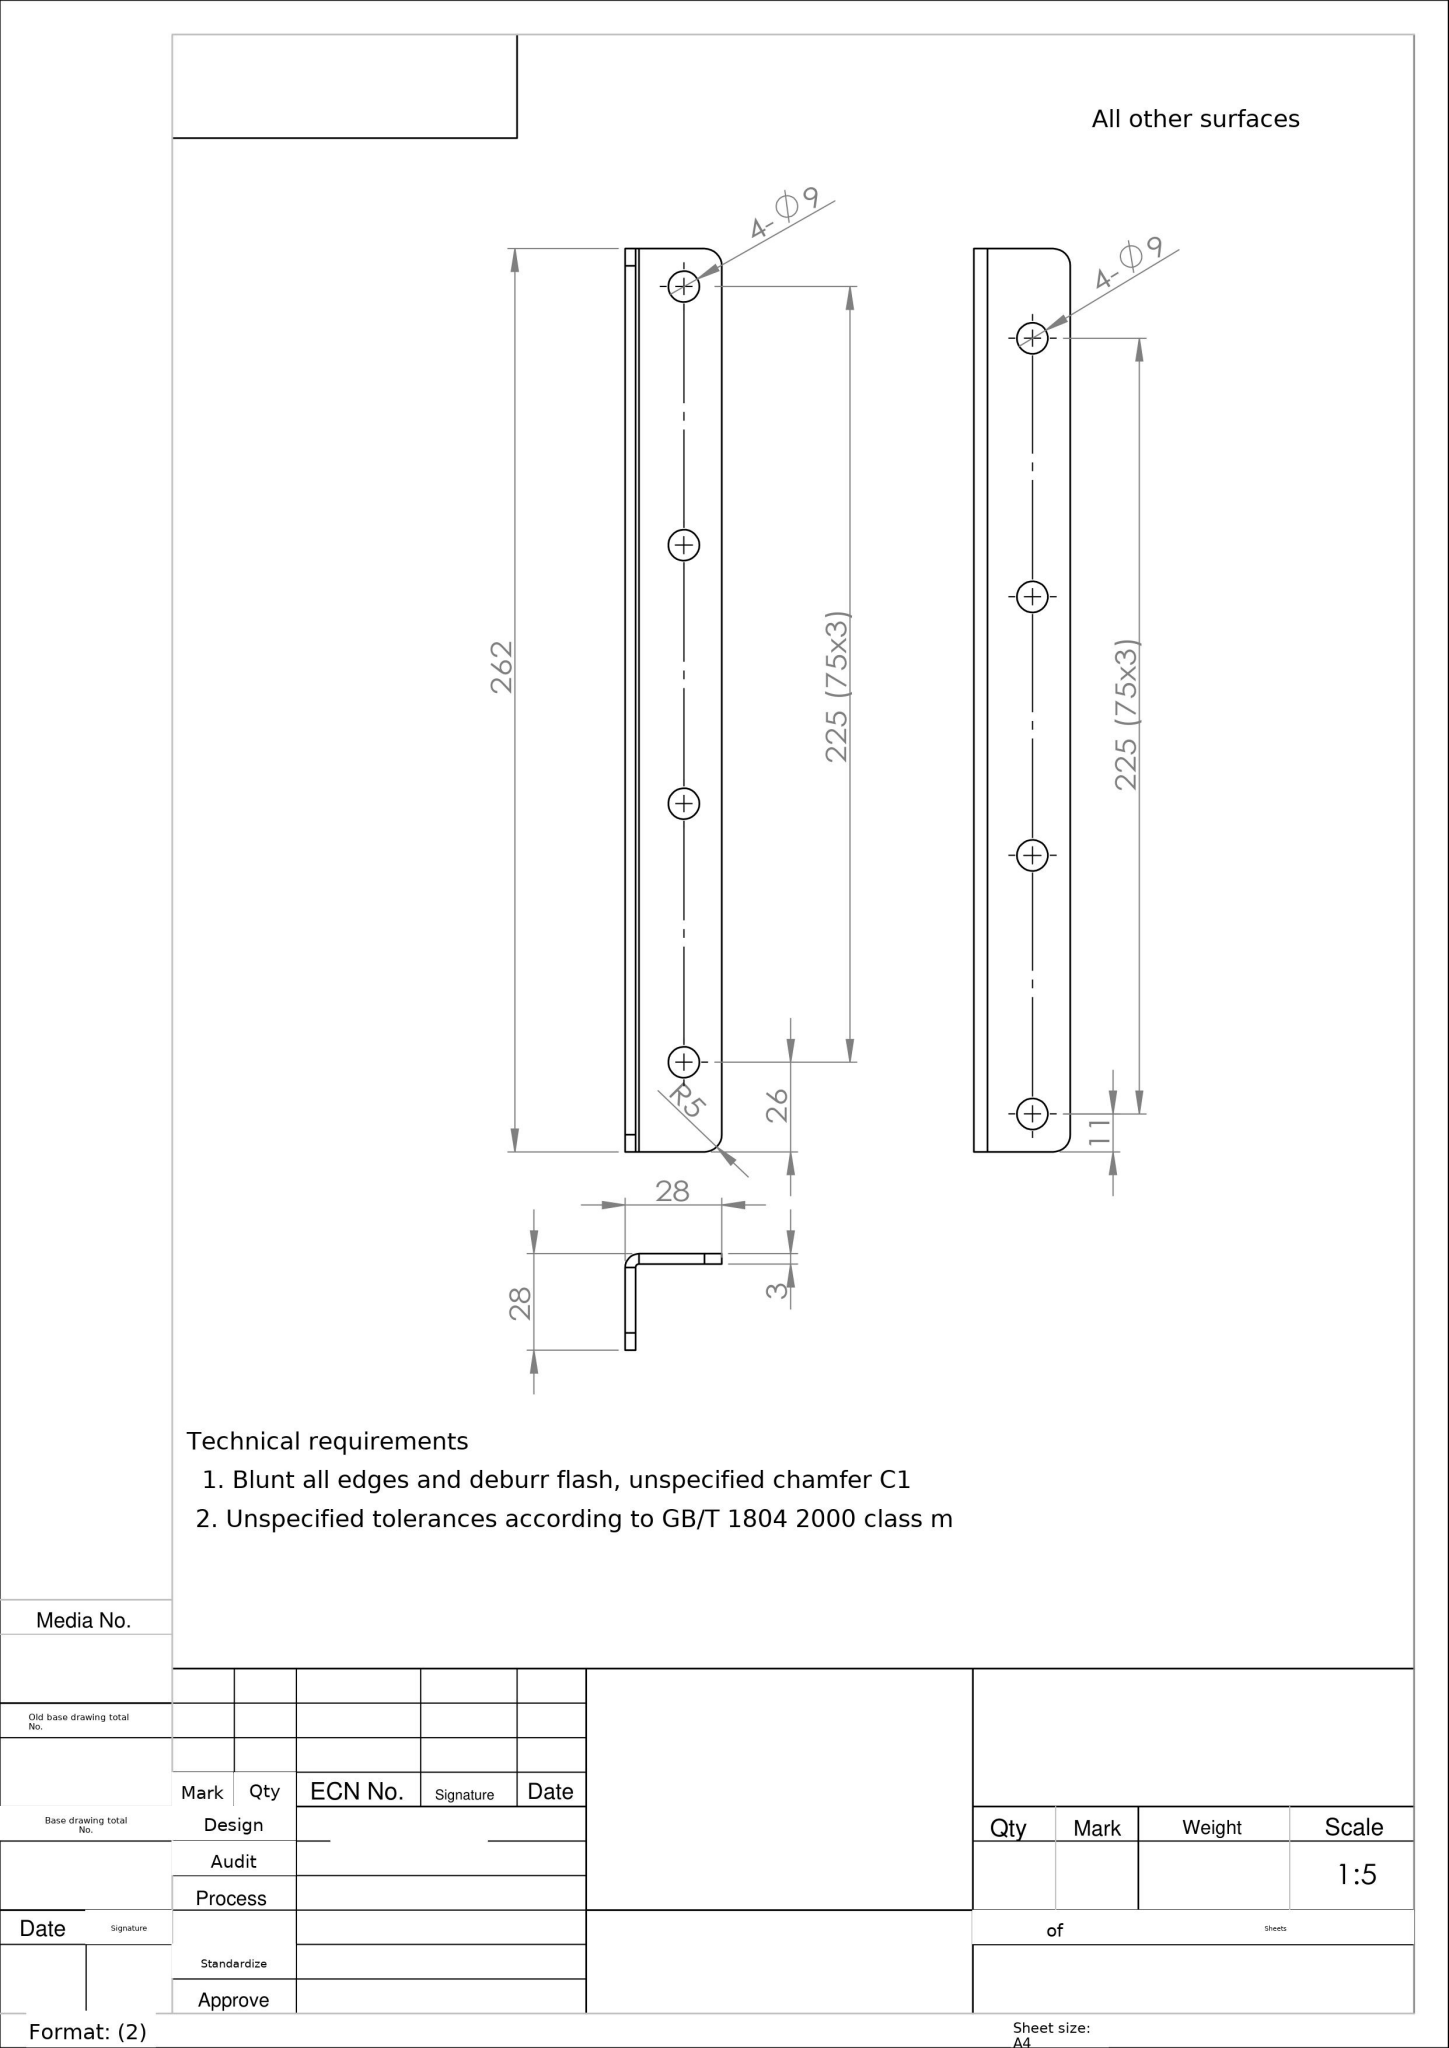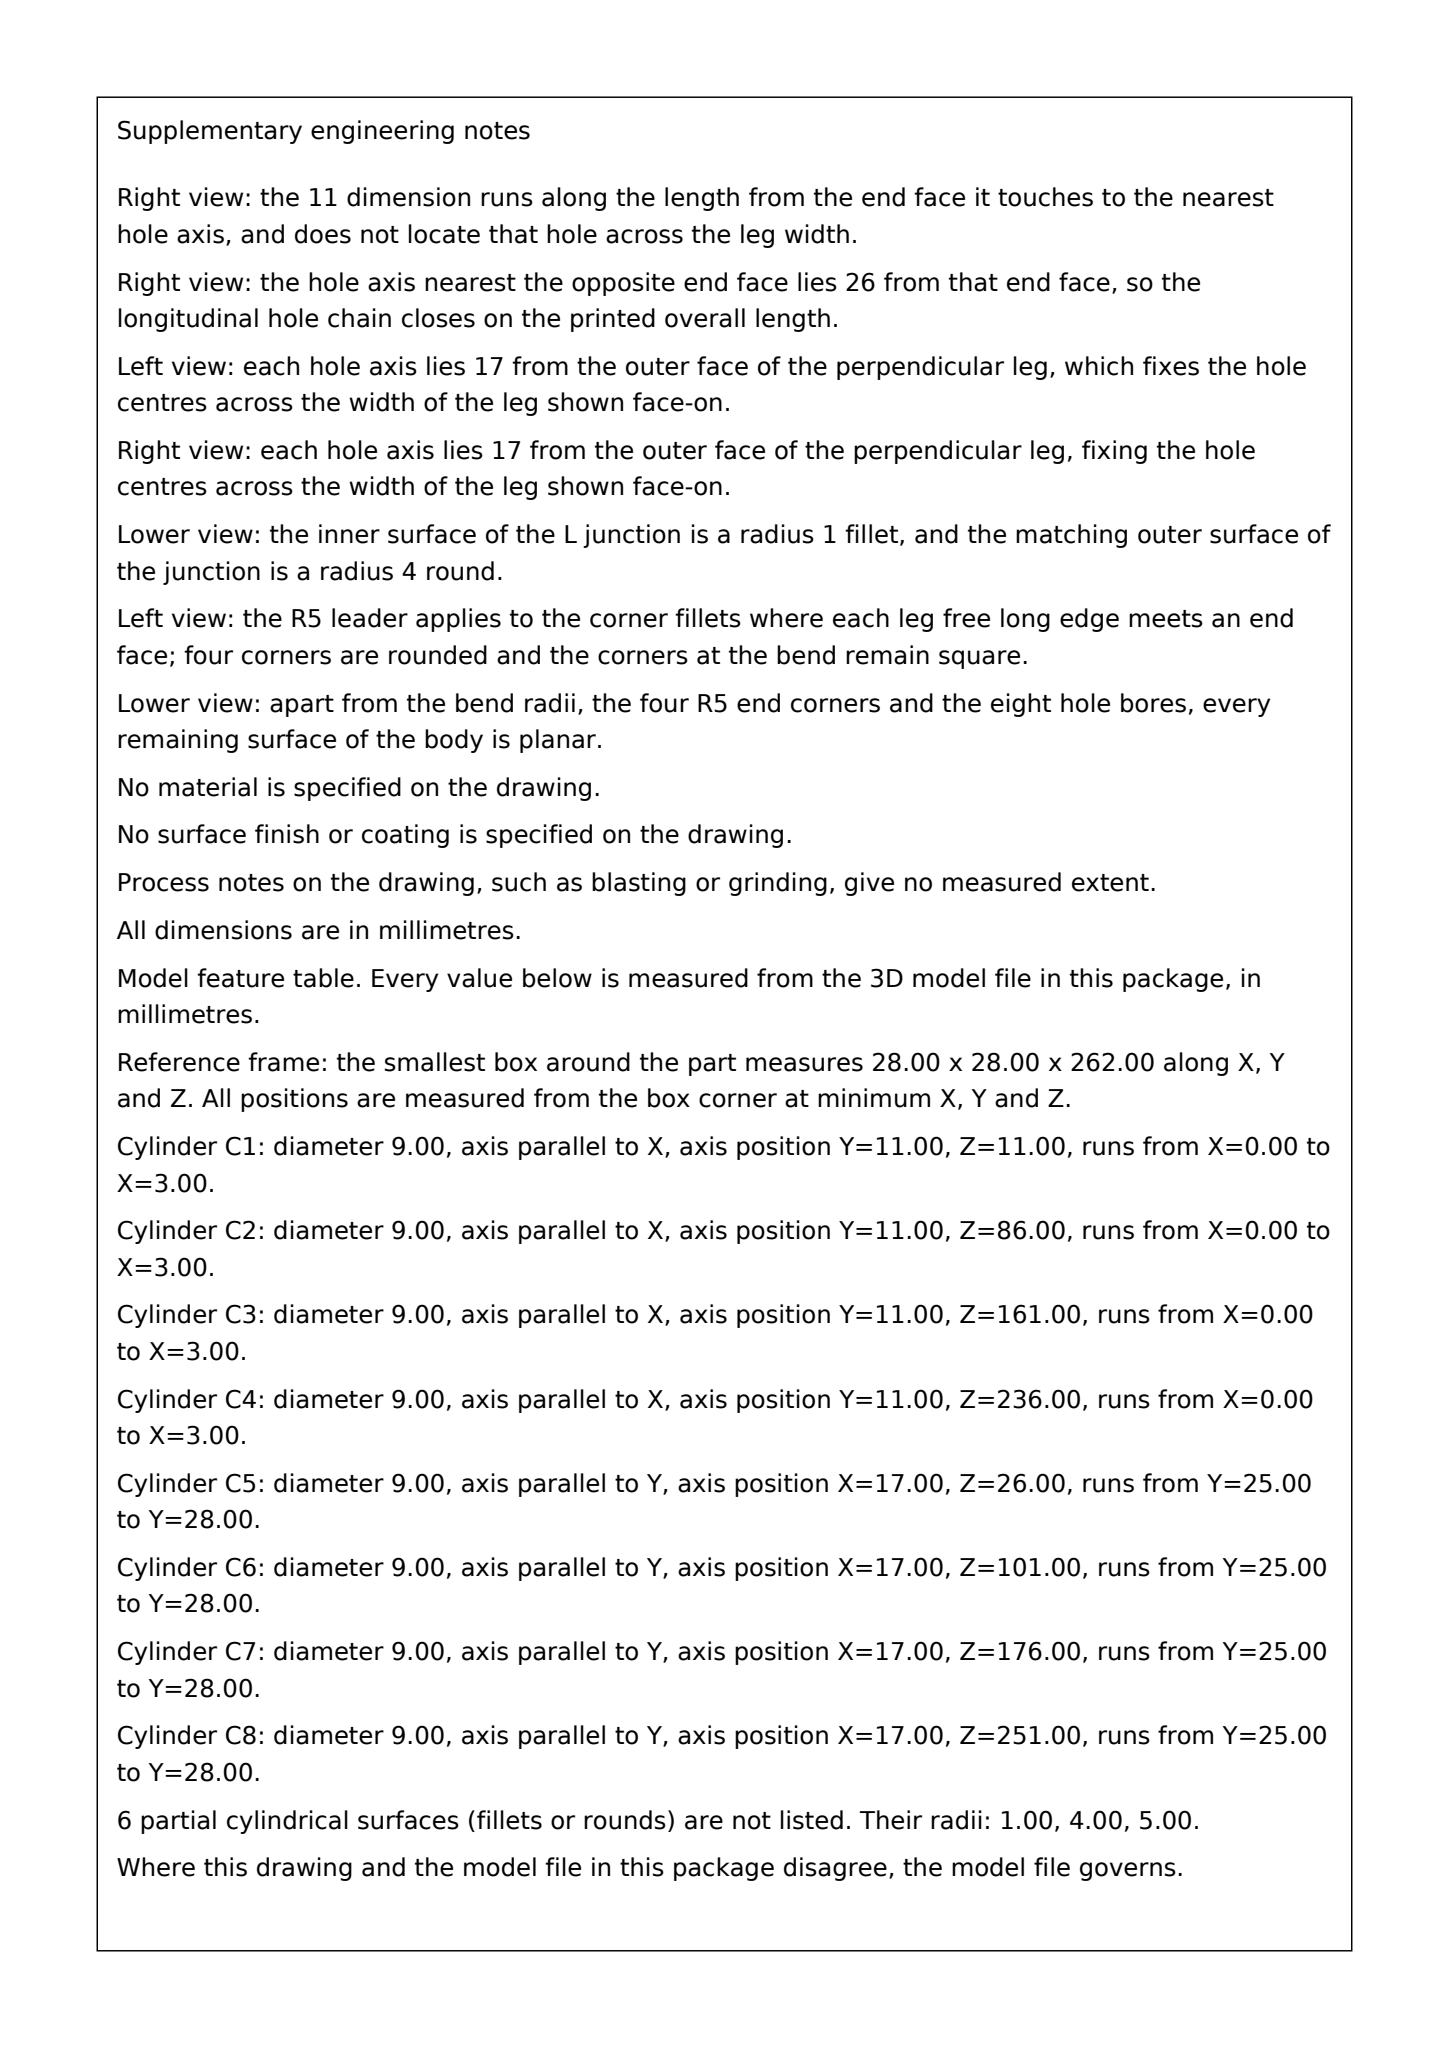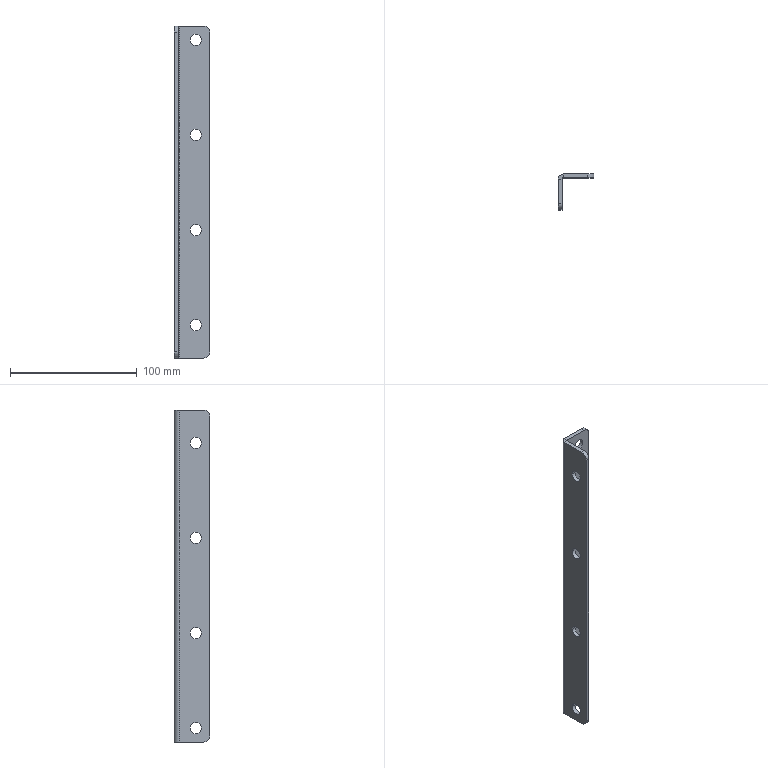Part | SolidWorks | mm | 1 solid | 34 faces | box 28 x 28 x 262 mm | volume 39223 mm3 | cylinder 22 | plane 12 | commonest cylinder face diameters 9 x16 10 x4 2 x1 8 x1
Drawing notes:
VIEW 1: 4-Ø9 HOLE CL 17 FROM OUTER FACE OF VERT LEG | from the solid: Ø9 holes, axis y, at x=17 (planes x=0 outer face, x=28 free edge)
VIEW 2: 4-Ø9 HOLE CL 17 FROM OUTER FACE OF HORIZ LEG | from the solid: Ø9 holes, axis x, at y=11; outer face plane y=28, so 28-11=17